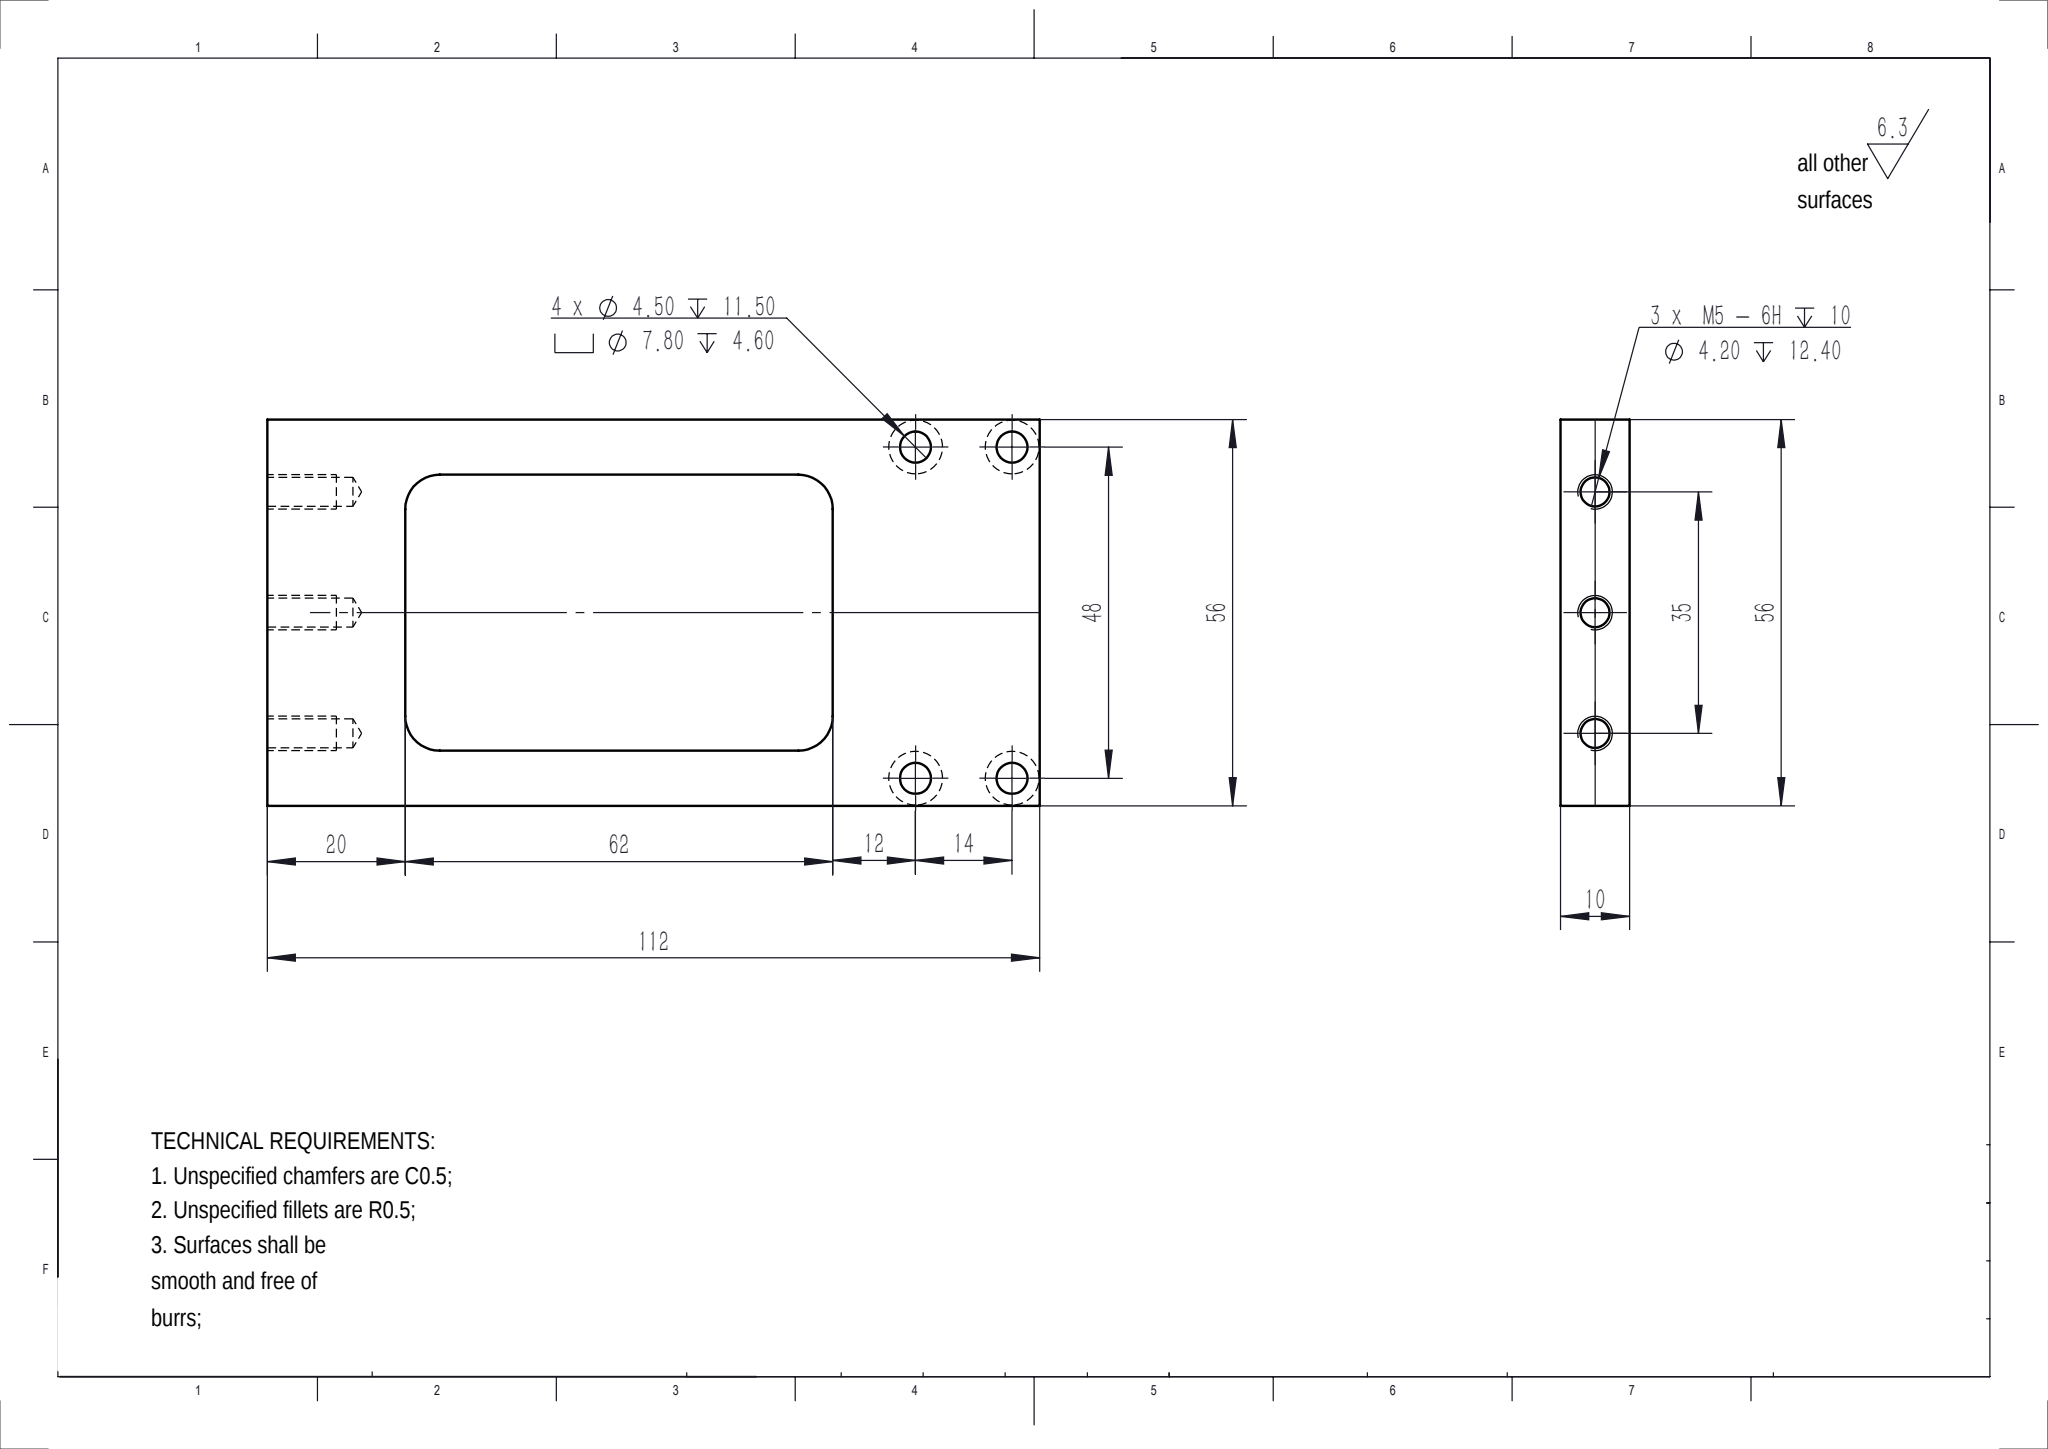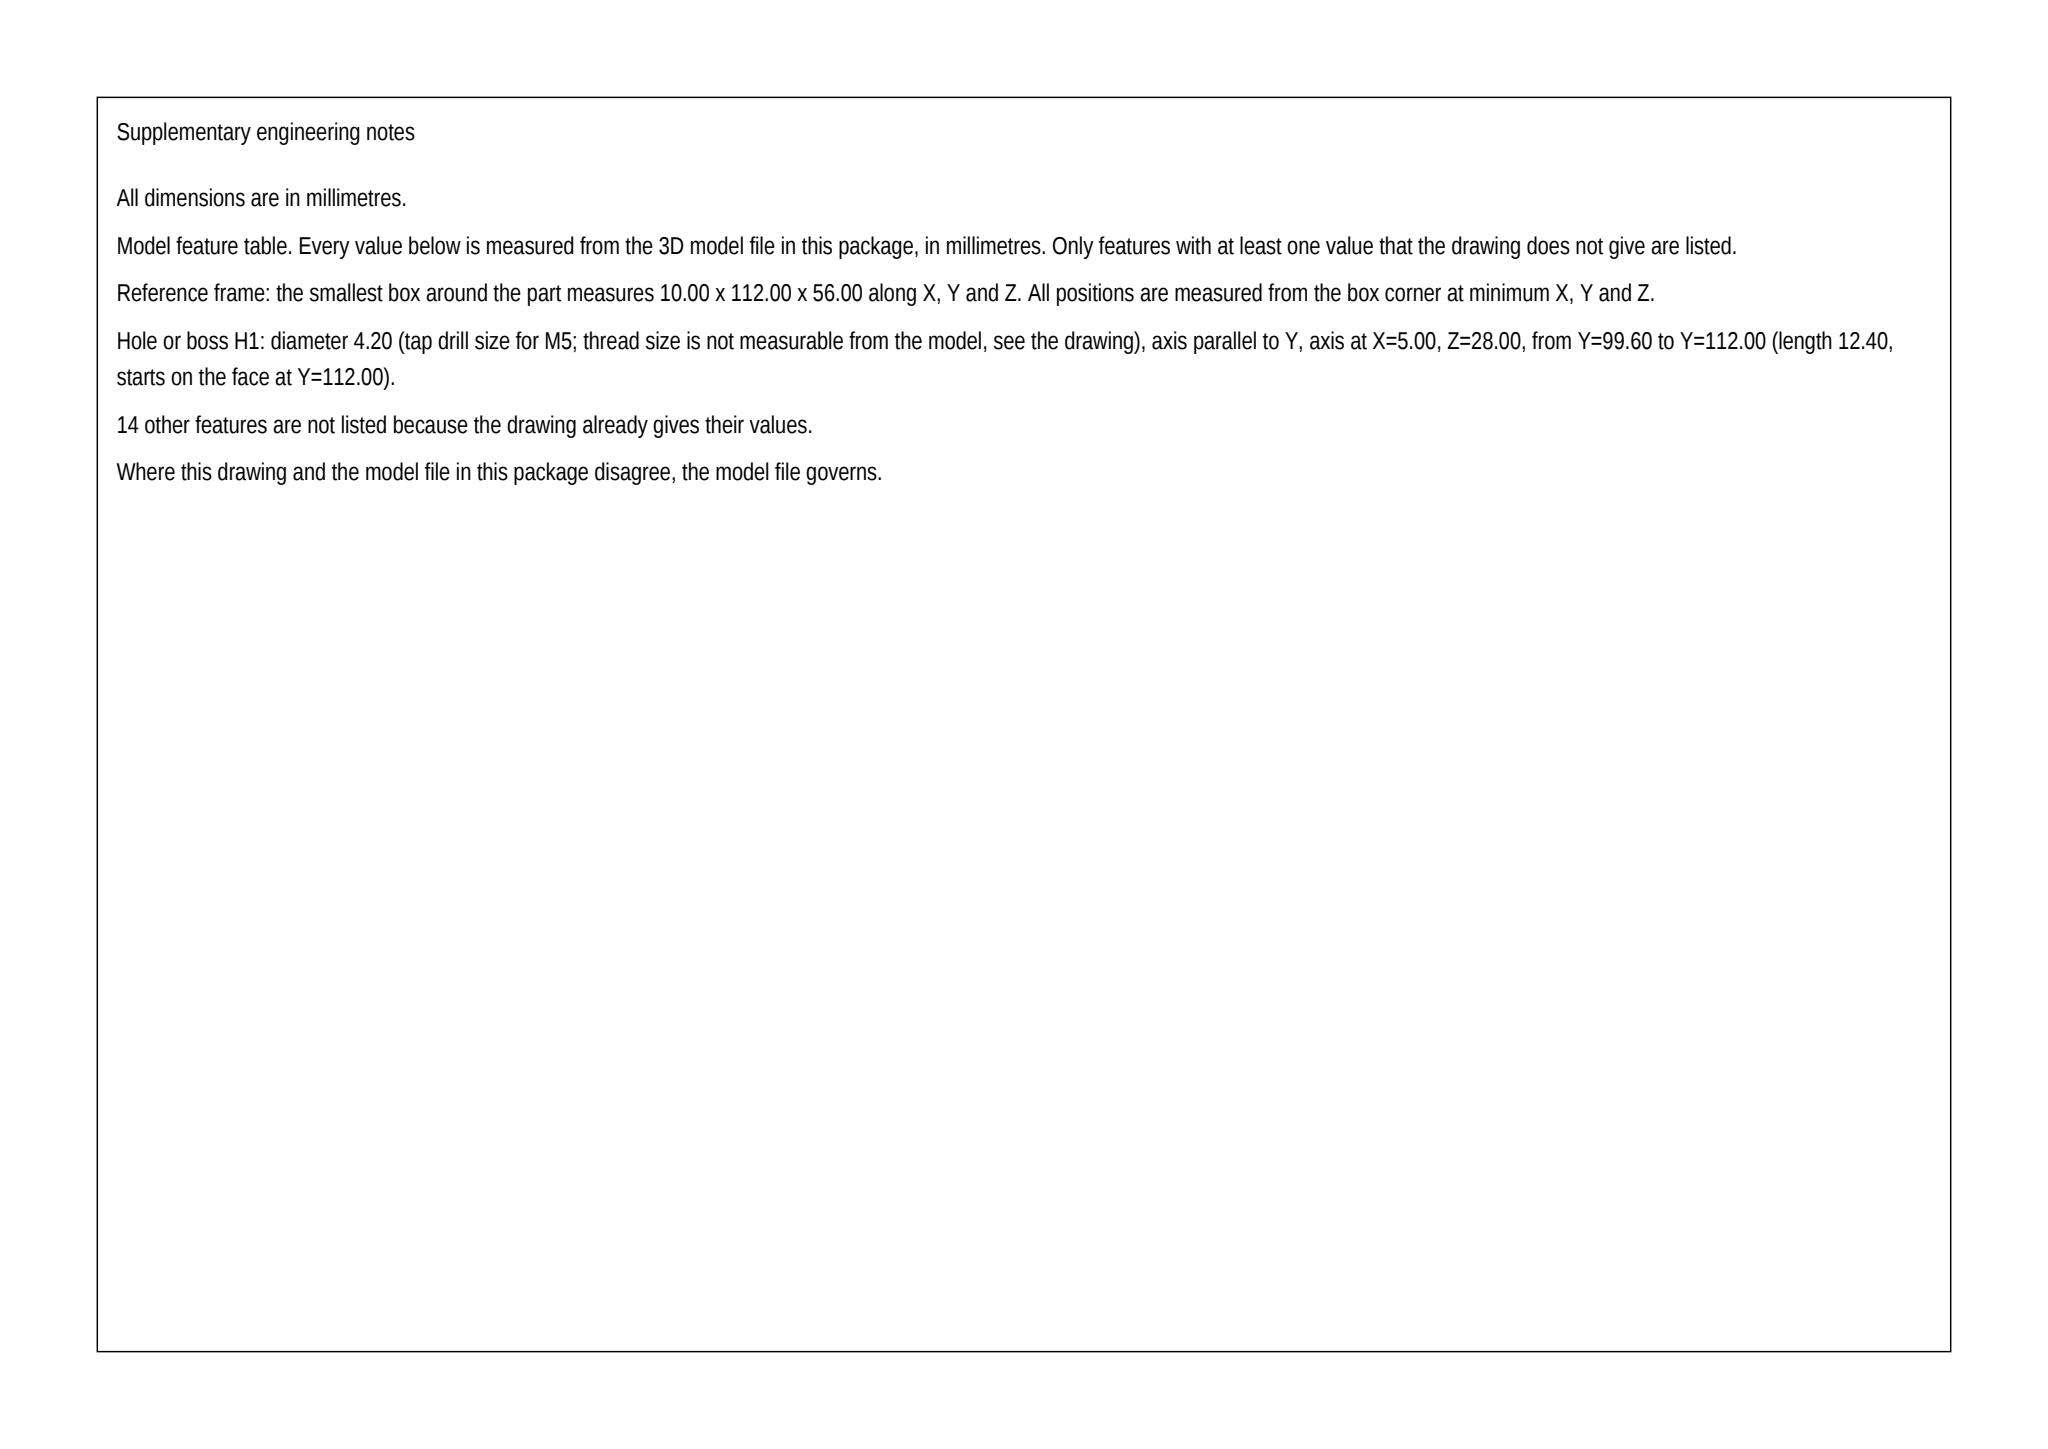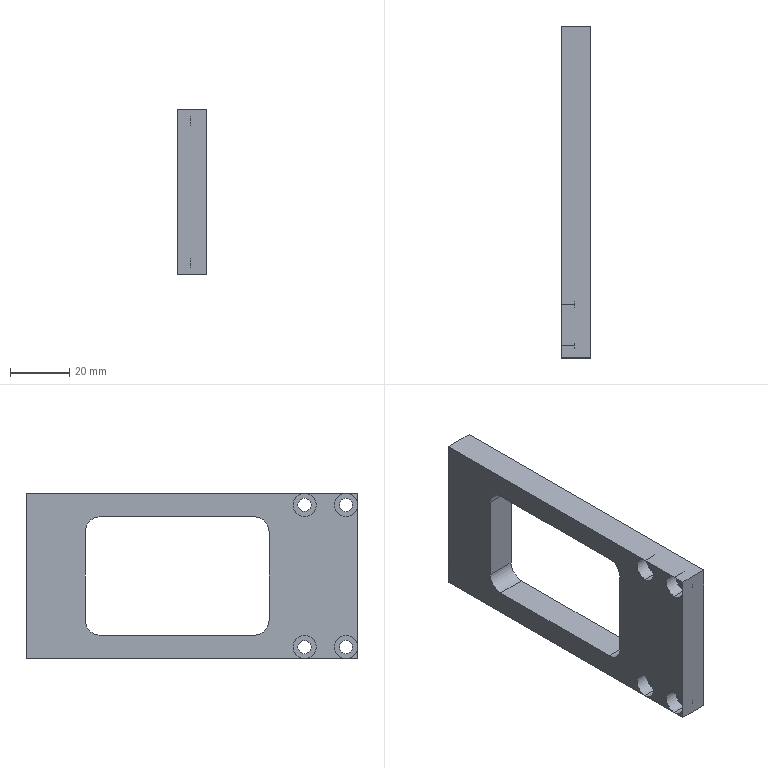Part | SolidWorks | mm | 1 solid | 46 faces | box 10 x 112 x 56 mm | volume 36379 mm3 | cylinder 26 | plane 14 | cone 6 | commonest cylinder face diameters 7.8 x8 4.5 x8 4.2 x6 10 x4
build123d program:
from build123d import *

# Parameters (mm, degrees)
SKETCH1_W                                         = 56
SKETCH1_H                                         = 112
BOSS_EXTRUDE1_DEPTH                               = 10
HOLE_SIZE_ACCORDING_TO_HEX_SOCKET_HEA_D           = 4.5
HOLE_SIZE_ACCORDING_TO_HEX_SOCKET_HEA_DEPTH       = 11.5
HOLE_SIZE_ACCORDING_TO_HEX_SOCKET_HEA_CBORE_D     = 7.8
HOLE_SIZE_ACCORDING_TO_HEX_SOCKET_HEA_CBORE_DEPTH = 4.6
HOLE_SIZE_ACCORDING_TO_HEX_SOCKET_HEA_TIP         = 1.352
M5_TAPPED_HOLE1_D                                 = 4.2
M5_TAPPED_HOLE1_DEPTH                             = 12.4
M5_TAPPED_HOLE1_TIP                               = 1.262
CUT_EXTRUDE1_DEPTH                                = 10


with BuildPart() as part:
    # Sketch1 → Boss-Extrude1 (new body)
    with BuildSketch(Plane(origin=(0, 0, 0), x_dir=(0, 0, -1), z_dir=(1, 0, 0))):
        Rectangle(SKETCH1_W, SKETCH1_H)
    extrude(amount=BOSS_EXTRUDE1_DEPTH)

    # Hole Size _ according to_ Hex Socket Hea
    with Locations(Plane.ZY):
        with Locations((-24, -52), (-24, -38), (24, -38), (24, -52)):
            CounterBoreHole(HOLE_SIZE_ACCORDING_TO_HEX_SOCKET_HEA_D / 2, HOLE_SIZE_ACCORDING_TO_HEX_SOCKET_HEA_CBORE_D / 2, HOLE_SIZE_ACCORDING_TO_HEX_SOCKET_HEA_CBORE_DEPTH, depth=HOLE_SIZE_ACCORDING_TO_HEX_SOCKET_HEA_DEPTH)
            with Locations((0, 0, -(HOLE_SIZE_ACCORDING_TO_HEX_SOCKET_HEA_DEPTH + HOLE_SIZE_ACCORDING_TO_HEX_SOCKET_HEA_TIP / 2))):  # 118° drill point
                Cone(0, HOLE_SIZE_ACCORDING_TO_HEX_SOCKET_HEA_D / 2, HOLE_SIZE_ACCORDING_TO_HEX_SOCKET_HEA_TIP, mode=Mode.SUBTRACT)

    # M5 Tapped Hole1
    with Locations(Plane(origin=(0, 56, 0), x_dir=(1, 0, 0), z_dir=(0, 1, 0))):
        with Locations((5, 17.5), (5, 0), (5, -17.5)):
            Hole(M5_TAPPED_HOLE1_D / 2, depth=M5_TAPPED_HOLE1_DEPTH)
            with Locations((0, 0, -(M5_TAPPED_HOLE1_DEPTH + M5_TAPPED_HOLE1_TIP / 2))):  # 118° drill point
                Cone(0, M5_TAPPED_HOLE1_D / 2, M5_TAPPED_HOLE1_TIP, mode=Mode.SUBTRACT)

    # Sketch6 → Cut-Extrude1 (cut)
    with BuildSketch(Plane.ZY):
        with BuildLine():
            Line((-15, 36), (15, 36))
            ThreePointArc((15, 36), (18.536, 34.536), (20, 31))
            Line((20, 31), (20, -21))
            ThreePointArc((20, -21), (18.536, -24.536), (15, -26))
            Line((15, -26), (-15, -26))
            ThreePointArc((-15, -26), (-18.536, -24.536), (-20, -21))
            Line((-20, -21), (-20, 31))
            ThreePointArc((-20, 31), (-18.536, 34.536), (-15, 36))
        make_face()
    extrude(amount=-CUT_EXTRUDE1_DEPTH, mode=Mode.SUBTRACT)


solid = part.part